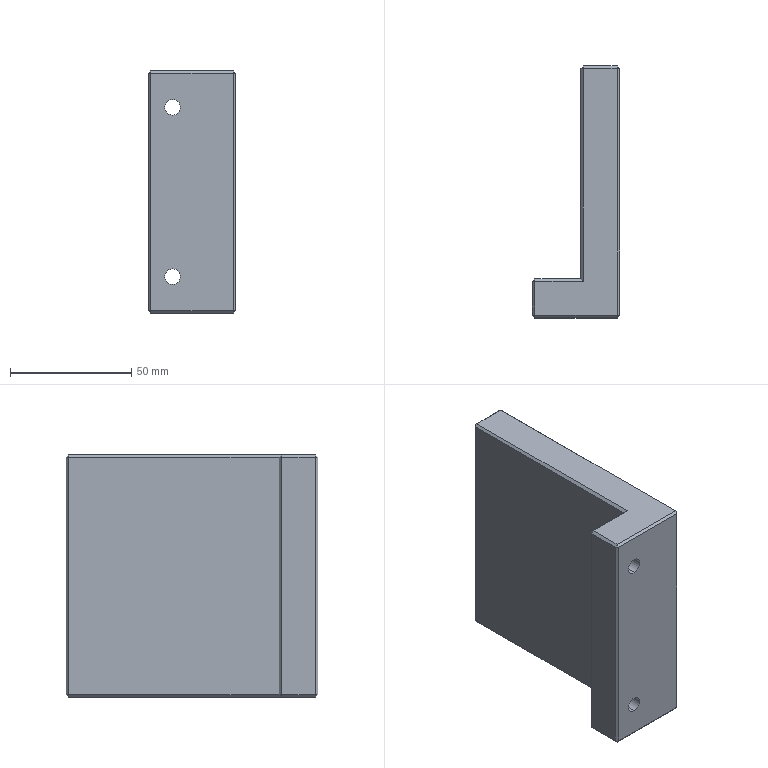Component | SolidWorks | GuideSupport-6 | 1 solid | 47 faces | box 36 x 104 x 100 mm | volume 196415 mm3 | plane 35 | cylinder 8 | cone 4 | commonest cylinder face diameters 4.2 x4 6.5 x4
build123d program:
from build123d import *

# Parameters (mm, degrees)
BOSS_EXTRUDE1_DEPTH   = 100
SKETCH2_R             = 3.25
CUT_EXTRUDE1_DEPTH    = 135.7
M5_TAPPED_HOLE1_D     = 4.2
M5_TAPPED_HOLE1_DEPTH = 14
M5_TAPPED_HOLE1_TIP   = 1.262
CHAMFER1_SIZE         = 1


with BuildPart() as part:
    # Sketch1 → Boss-Extrude1 (new body)
    with BuildSketch(Plane.XY):
        Polygon((0, 0), (0, -88), (-20, -88), (-20, -104), (16, -104), (16, 0), align=None)
    extrude(amount=BOSS_EXTRUDE1_DEPTH)

    # Sketch2 → Cut-Extrude1 (cut, through all)
    with BuildSketch(Plane(origin=(0, -88, 0), x_dir=(1, 0, 0), z_dir=(0, 1, 0))):
        with Locations(Location((-10, -15, 0), (0, 0, 270))):
            Circle(SKETCH2_R)
        with Locations(Location((-10, -85, 0), (0, 0, 270))):
            Circle(SKETCH2_R)
    extrude(amount=-CUT_EXTRUDE1_DEPTH, mode=Mode.SUBTRACT)

    # M5 Tapped Hole1
    with Locations(Plane(origin=(0, 0, 0), x_dir=(1, 0, 0), z_dir=(0, 1, 0))):
        with Locations((8, -15), (8, -85)):
            Hole(M5_TAPPED_HOLE1_D / 2, depth=M5_TAPPED_HOLE1_DEPTH)
            with Locations((0, 0, -(M5_TAPPED_HOLE1_DEPTH + M5_TAPPED_HOLE1_TIP / 2))):  # 118° drill point
                Cone(0, M5_TAPPED_HOLE1_D / 2, M5_TAPPED_HOLE1_TIP, mode=Mode.SUBTRACT)

    # Chamfer1
    chamfer1_edges = [part.edges().sort_by_distance(p)[0] for p in [
        (-10, -88, 100),
        (16, 0, 50),
        (16, -104, 50),
        (-20, -104, 50),
        (-20, -88, 50),
        (0, 0, 50),
        (-20, -96, 100),
        (-2, -104, 100),
        (16, -52, 100),
        (8, 0, 100),
        (16, -52, 0),
        (-2, -104, 0),
        (-20, -96, 0),
        (0, -44, 100),
        (-10, -88, 0),
        (0, -44, 0),
        (8, 0, 0),
    ]]
    chamfer(chamfer1_edges, length=CHAMFER1_SIZE)


solid = part.part

# Placed as in the assembly
solid = solid.moved(Location((-3.951, 421.323, 235), (0, 0, 0)))